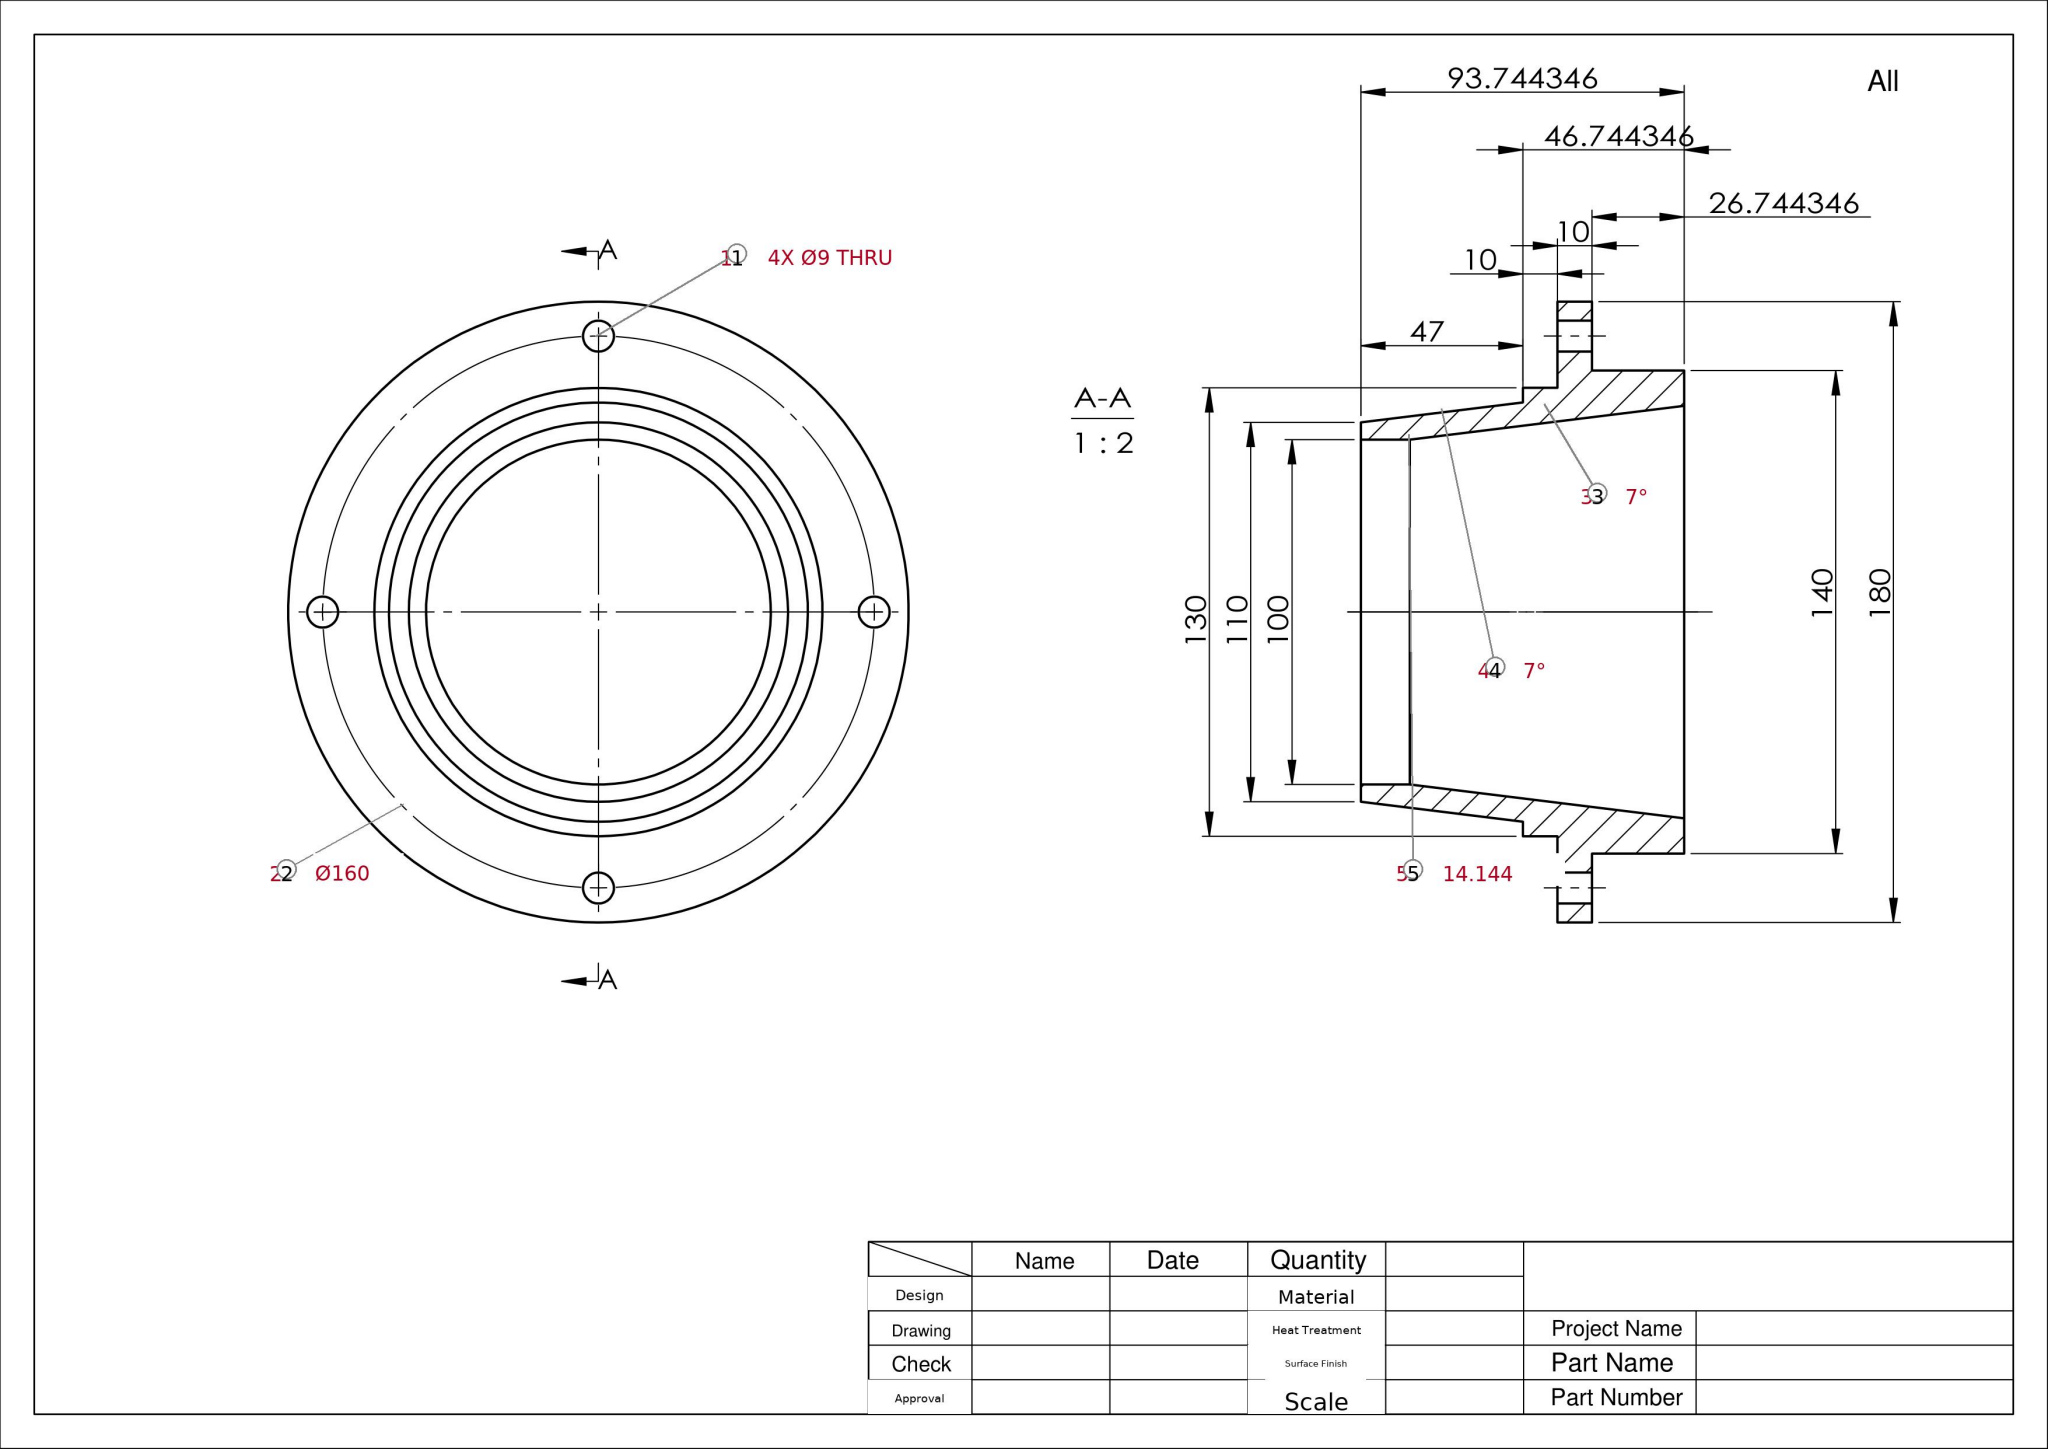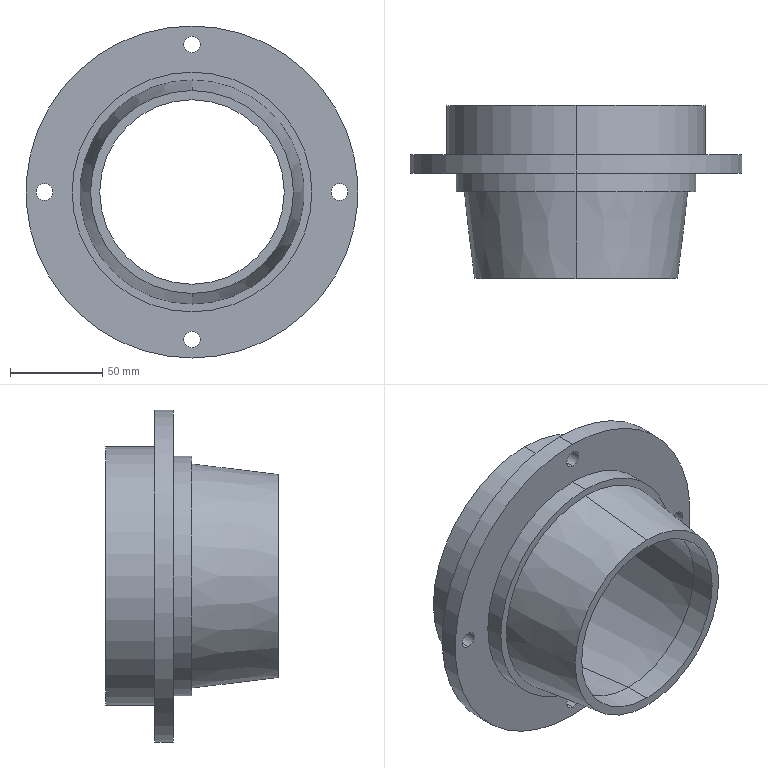Part | SolidWorks | mm | 1 solid | 25 faces | box 180 x 93.74 x 180 mm | volume 425080 mm3 | cylinder 16 | plane 5 | cone 4 | commonest cylinder face diameters 9 x8 180 x2 140 x2 100 x2 130 x2
STEP:
#1=CARTESIAN_POINT('',(0.,-6.,-55.));
#2=VERTEX_POINT('',#1);
#3=CARTESIAN_POINT('',(0.,-6.,55.));
#4=VERTEX_POINT('',#3);
#5=CARTESIAN_POINT('',(0.,-6.,0.));
#6=DIRECTION('',(0.,-1.,0.));
#7=DIRECTION('',(0.,0.,-1.));
#8=AXIS2_PLACEMENT_3D('',#5,#6,#7);
#9=CIRCLE('',#8,55.);
#10=EDGE_CURVE('',#2,#4,#9,.T.);
#11=ORIENTED_EDGE('',*,*,#10,.F.);
#12=CARTESIAN_POINT('',(0.,41.,-60.771));
#13=VERTEX_POINT('',#12);
#14=CARTESIAN_POINT('',(0.,41.,-60.771));
#15=DIRECTION('',(0.,0.9925,-0.1219));
#16=VECTOR('',#15,1000.);
#17=LINE('',#14,#16);
#18=EDGE_CURVE('',#2,#13,#17,.T.);
#19=ORIENTED_EDGE('',*,*,#18,.T.);
#20=CARTESIAN_POINT('',(0.,41.,60.771));
#21=VERTEX_POINT('',#20);
#22=CARTESIAN_POINT('',(0.,41.,0.));
#23=DIRECTION('',(0.,-1.,0.));
#24=DIRECTION('',(0.,0.,-1.));
#25=AXIS2_PLACEMENT_3D('',#22,#23,#24);
#26=CIRCLE('',#25,60.771);
#27=EDGE_CURVE('',#13,#21,#26,.T.);
#28=ORIENTED_EDGE('',*,*,#27,.T.);
#29=CARTESIAN_POINT('',(0.,41.,60.771));
#30=DIRECTION('',(0.,0.9925,0.1219));
#31=VECTOR('',#30,1000.);
#32=LINE('',#29,#31);
#33=EDGE_CURVE('',#4,#21,#32,.T.);
#34=ORIENTED_EDGE('',*,*,#33,.F.);
#35=EDGE_LOOP('',(#11,#19,#28,#34));
#36=FACE_OUTER_BOUND('',#35,.T.);
#37=CARTESIAN_POINT('',(0.,41.,0.));
#38=DIRECTION('',(0.,1.,0.));
#39=DIRECTION('',(0.,0.,1.));
#40=AXIS2_PLACEMENT_3D('',#37,#38,#39);
#41=CONICAL_SURFACE('',#40,60.771,0.1222);
#42=ADVANCED_FACE('',(#36),#41,.T.);
#43=CARTESIAN_POINT('',(80.,51.,4.5));
#44=VERTEX_POINT('',#43);
#45=CARTESIAN_POINT('',(80.,51.,-4.5));
#46=VERTEX_POINT('',#45);
#47=CARTESIAN_POINT('',(80.,51.,-0.));
#48=DIRECTION('',(0.,-1.,0.));
#49=DIRECTION('',(0.,0.,-1.));
#50=AXIS2_PLACEMENT_3D('',#47,#48,#49);
#51=CIRCLE('',#50,4.5);
#52=EDGE_CURVE('',#44,#46,#51,.T.);
#53=ORIENTED_EDGE('',*,*,#52,.T.);
#54=CARTESIAN_POINT('',(80.,61.,-4.5));
#55=VERTEX_POINT('',#54);
#56=CARTESIAN_POINT('',(80.,-10.,-4.5));
#57=DIRECTION('',(0.,1.,0.));
#58=VECTOR('',#57,1000.);
#59=LINE('',#56,#58);
#60=EDGE_CURVE('',#46,#55,#59,.T.);
#61=ORIENTED_EDGE('',*,*,#60,.T.);
#62=CARTESIAN_POINT('',(80.,61.,4.5));
#63=VERTEX_POINT('',#62);
#64=CARTESIAN_POINT('',(80.,61.,-0.));
#65=DIRECTION('',(0.,1.,0.));
#66=DIRECTION('',(-1.,0.,0.));
#67=AXIS2_PLACEMENT_3D('',#64,#65,#66);
#68=CIRCLE('',#67,4.5);
#69=EDGE_CURVE('',#55,#63,#68,.T.);
#70=ORIENTED_EDGE('',*,*,#69,.T.);
#71=CARTESIAN_POINT('',(80.,-10.,4.5));
#72=DIRECTION('',(0.,1.,0.));
#73=VECTOR('',#72,1000.);
#74=LINE('',#71,#73);
#75=EDGE_CURVE('',#44,#63,#74,.T.);
#76=ORIENTED_EDGE('',*,*,#75,.F.);
#77=EDGE_LOOP('',(#53,#61,#70,#76));
#78=FACE_OUTER_BOUND('',#77,.T.);
#79=CARTESIAN_POINT('',(80.,-10.,-0.));
#80=DIRECTION('',(0.,1.,0.));
#81=DIRECTION('',(0.,0.,1.));
#82=AXIS2_PLACEMENT_3D('',#79,#80,#81);
#83=CYLINDRICAL_SURFACE('',#82,4.5);
#84=ADVANCED_FACE('',(#78),#83,.F.);
#85=CARTESIAN_POINT('',(0.,51.,84.5));
#86=VERTEX_POINT('',#85);
#87=CARTESIAN_POINT('',(0.,51.,75.5));
#88=VERTEX_POINT('',#87);
#89=CARTESIAN_POINT('',(0.,51.,80.));
#90=DIRECTION('',(0.,-1.,0.));
#91=DIRECTION('',(0.,0.,-1.));
#92=AXIS2_PLACEMENT_3D('',#89,#90,#91);
#93=CIRCLE('',#92,4.5);
#94=EDGE_CURVE('',#86,#88,#93,.T.);
#95=ORIENTED_EDGE('',*,*,#94,.T.);
#96=CARTESIAN_POINT('',(0.,61.,75.5));
#97=VERTEX_POINT('',#96);
#98=CARTESIAN_POINT('',(0.,-10.,75.5));
#99=DIRECTION('',(0.,1.,0.));
#100=VECTOR('',#99,1000.);
#101=LINE('',#98,#100);
#102=EDGE_CURVE('',#88,#97,#101,.T.);
#103=ORIENTED_EDGE('',*,*,#102,.T.);
#104=CARTESIAN_POINT('',(0.,61.,84.5));
#105=VERTEX_POINT('',#104);
#106=CARTESIAN_POINT('',(0.,61.,80.));
#107=DIRECTION('',(0.,1.,0.));
#108=DIRECTION('',(-0.,0.,-1.));
#109=AXIS2_PLACEMENT_3D('',#106,#107,#108);
#110=CIRCLE('',#109,4.5);
#111=EDGE_CURVE('',#97,#105,#110,.T.);
#112=ORIENTED_EDGE('',*,*,#111,.T.);
#113=CARTESIAN_POINT('',(0.,-10.,84.5));
#114=DIRECTION('',(0.,1.,0.));
#115=VECTOR('',#114,1000.);
#116=LINE('',#113,#115);
#117=EDGE_CURVE('',#86,#105,#116,.T.);
#118=ORIENTED_EDGE('',*,*,#117,.F.);
#119=EDGE_LOOP('',(#95,#103,#112,#118));
#120=FACE_OUTER_BOUND('',#119,.T.);
#121=CARTESIAN_POINT('',(0.,-10.,80.));
#122=DIRECTION('',(0.,1.,0.));
#123=DIRECTION('',(0.,0.,1.));
#124=AXIS2_PLACEMENT_3D('',#121,#122,#123);
#125=CYLINDRICAL_SURFACE('',#124,4.5);
#126=ADVANCED_FACE('',(#120),#125,.F.);
#127=CARTESIAN_POINT('',(-80.,51.,4.5));
#128=VERTEX_POINT('',#127);
#129=CARTESIAN_POINT('',(-80.,51.,-4.5));
#130=VERTEX_POINT('',#129);
#131=CARTESIAN_POINT('',(-80.,51.,0.));
#132=DIRECTION('',(0.,-1.,0.));
#133=DIRECTION('',(0.,0.,-1.));
#134=AXIS2_PLACEMENT_3D('',#131,#132,#133);
#135=CIRCLE('',#134,4.5);
#136=EDGE_CURVE('',#128,#130,#135,.T.);
#137=ORIENTED_EDGE('',*,*,#136,.T.);
#138=CARTESIAN_POINT('',(-80.,61.,-4.5));
#139=VERTEX_POINT('',#138);
#140=CARTESIAN_POINT('',(-80.,-10.,-4.5));
#141=DIRECTION('',(0.,1.,0.));
#142=VECTOR('',#141,1000.);
#143=LINE('',#140,#142);
#144=EDGE_CURVE('',#130,#139,#143,.T.);
#145=ORIENTED_EDGE('',*,*,#144,.T.);
#146=CARTESIAN_POINT('',(-80.,61.,4.5));
#147=VERTEX_POINT('',#146);
#148=CARTESIAN_POINT('',(-80.,61.,0.));
#149=DIRECTION('',(0.,1.,0.));
#150=DIRECTION('',(1.,0.,-0.));
#151=AXIS2_PLACEMENT_3D('',#148,#149,#150);
#152=CIRCLE('',#151,4.5);
#153=EDGE_CURVE('',#139,#147,#152,.T.);
#154=ORIENTED_EDGE('',*,*,#153,.T.);
#155=CARTESIAN_POINT('',(-80.,-10.,4.5));
#156=DIRECTION('',(0.,1.,0.));
#157=VECTOR('',#156,1000.);
#158=LINE('',#155,#157);
#159=EDGE_CURVE('',#128,#147,#158,.T.);
#160=ORIENTED_EDGE('',*,*,#159,.F.);
#161=EDGE_LOOP('',(#137,#145,#154,#160));
#162=FACE_OUTER_BOUND('',#161,.T.);
#163=CARTESIAN_POINT('',(-80.,-10.,0.));
#164=DIRECTION('',(0.,1.,0.));
#165=DIRECTION('',(0.,0.,1.));
#166=AXIS2_PLACEMENT_3D('',#163,#164,#165);
#167=CYLINDRICAL_SURFACE('',#166,4.5);
#168=ADVANCED_FACE('',(#162),#167,.F.);
#169=CARTESIAN_POINT('',(0.,51.,-75.5));
#170=VERTEX_POINT('',#169);
#171=CARTESIAN_POINT('',(0.,51.,-84.5));
#172=VERTEX_POINT('',#171);
#173=CARTESIAN_POINT('',(0.,51.,-80.));
#174=DIRECTION('',(0.,-1.,0.));
#175=DIRECTION('',(0.,0.,-1.));
#176=AXIS2_PLACEMENT_3D('',#173,#174,#175);
#177=CIRCLE('',#176,4.5);
#178=EDGE_CURVE('',#170,#172,#177,.T.);
#179=ORIENTED_EDGE('',*,*,#178,.T.);
#180=CARTESIAN_POINT('',(0.,61.,-84.5));
#181=VERTEX_POINT('',#180);
#182=CARTESIAN_POINT('',(0.,-10.,-84.5));
#183=DIRECTION('',(0.,1.,0.));
#184=VECTOR('',#183,1000.);
#185=LINE('',#182,#184);
#186=EDGE_CURVE('',#172,#181,#185,.T.);
#187=ORIENTED_EDGE('',*,*,#186,.T.);
#188=CARTESIAN_POINT('',(0.,61.,-75.5));
#189=VERTEX_POINT('',#188);
#190=CARTESIAN_POINT('',(0.,61.,-80.));
#191=DIRECTION('',(0.,1.,0.));
#192=DIRECTION('',(0.,0.,1.));
#193=AXIS2_PLACEMENT_3D('',#190,#191,#192);
#194=CIRCLE('',#193,4.5);
#195=EDGE_CURVE('',#181,#189,#194,.T.);
#196=ORIENTED_EDGE('',*,*,#195,.T.);
#197=CARTESIAN_POINT('',(0.,-10.,-75.5));
#198=DIRECTION('',(0.,1.,0.));
#199=VECTOR('',#198,1000.);
#200=LINE('',#197,#199);
#201=EDGE_CURVE('',#170,#189,#200,.T.);
#202=ORIENTED_EDGE('',*,*,#201,.F.);
#203=EDGE_LOOP('',(#179,#187,#196,#202));
#204=FACE_OUTER_BOUND('',#203,.T.);
#205=CARTESIAN_POINT('',(0.,-10.,-80.));
#206=DIRECTION('',(0.,1.,0.));
#207=DIRECTION('',(0.,0.,1.));
#208=AXIS2_PLACEMENT_3D('',#205,#206,#207);
#209=CYLINDRICAL_SURFACE('',#208,4.5);
#210=ADVANCED_FACE('',(#204),#209,.F.);
#211=CARTESIAN_POINT('',(0.,51.,-90.));
#212=VERTEX_POINT('',#211);
#213=CARTESIAN_POINT('',(0.,51.,90.));
#214=VERTEX_POINT('',#213);
#215=CARTESIAN_POINT('',(0.,51.,0.));
#216=DIRECTION('',(0.,-1.,0.));
#217=DIRECTION('',(0.,0.,-1.));
#218=AXIS2_PLACEMENT_3D('',#215,#216,#217);
#219=CIRCLE('',#218,90.);
#220=EDGE_CURVE('',#212,#214,#219,.T.);
#221=ORIENTED_EDGE('',*,*,#220,.F.);
#222=CARTESIAN_POINT('',(0.,61.,-90.));
#223=VERTEX_POINT('',#222);
#224=CARTESIAN_POINT('',(0.,-10.,-90.));
#225=DIRECTION('',(0.,1.,0.));
#226=VECTOR('',#225,1000.);
#227=LINE('',#224,#226);
#228=EDGE_CURVE('',#212,#223,#227,.T.);
#229=ORIENTED_EDGE('',*,*,#228,.T.);
#230=CARTESIAN_POINT('',(0.,61.,90.));
#231=VERTEX_POINT('',#230);
#232=CARTESIAN_POINT('',(0.,61.,0.));
#233=DIRECTION('',(0.,1.,0.));
#234=DIRECTION('',(0.,0.,1.));
#235=AXIS2_PLACEMENT_3D('',#232,#233,#234);
#236=CIRCLE('',#235,90.);
#237=EDGE_CURVE('',#231,#223,#236,.T.);
#238=ORIENTED_EDGE('',*,*,#237,.F.);
#239=CARTESIAN_POINT('',(0.,-10.,90.));
#240=DIRECTION('',(0.,1.,0.));
#241=VECTOR('',#240,1000.);
#242=LINE('',#239,#241);
#243=EDGE_CURVE('',#214,#231,#242,.T.);
#244=ORIENTED_EDGE('',*,*,#243,.F.);
#245=EDGE_LOOP('',(#221,#229,#238,#244));
#246=FACE_OUTER_BOUND('',#245,.T.);
#247=CARTESIAN_POINT('',(0.,-10.,0.));
#248=DIRECTION('',(0.,1.,0.));
#249=DIRECTION('',(0.,0.,1.));
#250=AXIS2_PLACEMENT_3D('',#247,#248,#249);
#251=CYLINDRICAL_SURFACE('',#250,90.);
#252=ADVANCED_FACE('',(#246),#251,.T.);
#253=CARTESIAN_POINT('',(0.,61.,-70.));
#254=VERTEX_POINT('',#253);
#255=CARTESIAN_POINT('',(0.,61.,70.));
#256=VERTEX_POINT('',#255);
#257=CARTESIAN_POINT('',(0.,61.,0.));
#258=DIRECTION('',(0.,-1.,0.));
#259=DIRECTION('',(0.,0.,1.));
#260=AXIS2_PLACEMENT_3D('',#257,#258,#259);
#261=CIRCLE('',#260,70.);
#262=EDGE_CURVE('',#254,#256,#261,.T.);
#263=ORIENTED_EDGE('',*,*,#262,.F.);
#264=CARTESIAN_POINT('',(0.,87.744,-70.));
#265=VERTEX_POINT('',#264);
#266=CARTESIAN_POINT('',(0.,-191.367,-70.));
#267=DIRECTION('',(0.,1.,0.));
#268=VECTOR('',#267,1000.);
#269=LINE('',#266,#268);
#270=EDGE_CURVE('',#254,#265,#269,.T.);
#271=ORIENTED_EDGE('',*,*,#270,.T.);
#272=CARTESIAN_POINT('',(0.,87.744,70.));
#273=VERTEX_POINT('',#272);
#274=CARTESIAN_POINT('',(0.,87.744,0.));
#275=DIRECTION('',(0.,-1.,0.));
#276=DIRECTION('',(0.,0.,-1.));
#277=AXIS2_PLACEMENT_3D('',#274,#275,#276);
#278=CIRCLE('',#277,70.);
#279=EDGE_CURVE('',#265,#273,#278,.T.);
#280=ORIENTED_EDGE('',*,*,#279,.T.);
#281=CARTESIAN_POINT('',(0.,-191.367,70.));
#282=DIRECTION('',(0.,1.,0.));
#283=VECTOR('',#282,1000.);
#284=LINE('',#281,#283);
#285=EDGE_CURVE('',#256,#273,#284,.T.);
#286=ORIENTED_EDGE('',*,*,#285,.F.);
#287=EDGE_LOOP('',(#263,#271,#280,#286));
#288=FACE_OUTER_BOUND('',#287,.T.);
#289=CARTESIAN_POINT('',(0.,-191.367,0.));
#290=DIRECTION('',(0.,1.,0.));
#291=DIRECTION('',(0.,0.,1.));
#292=AXIS2_PLACEMENT_3D('',#289,#290,#291);
#293=CYLINDRICAL_SURFACE('',#292,70.);
#294=ADVANCED_FACE('',(#288),#293,.T.);
#295=CARTESIAN_POINT('',(0.,8.144,-50.));
#296=VERTEX_POINT('',#295);
#297=CARTESIAN_POINT('',(0.,8.144,50.));
#298=VERTEX_POINT('',#297);
#299=CARTESIAN_POINT('',(0.,8.144,0.));
#300=DIRECTION('',(0.,1.,0.));
#301=DIRECTION('',(0.,0.,1.));
#302=AXIS2_PLACEMENT_3D('',#299,#300,#301);
#303=CIRCLE('',#302,50.);
#304=EDGE_CURVE('',#296,#298,#303,.T.);
#305=ORIENTED_EDGE('',*,*,#304,.T.);
#306=CARTESIAN_POINT('',(0.,-6.,50.));
#307=VERTEX_POINT('',#306);
#308=CARTESIAN_POINT('',(0.,86.,50.));
#309=DIRECTION('',(0.,-1.,0.));
#310=VECTOR('',#309,1000.);
#311=LINE('',#308,#310);
#312=EDGE_CURVE('',#298,#307,#311,.T.);
#313=ORIENTED_EDGE('',*,*,#312,.T.);
#314=CARTESIAN_POINT('',(0.,-6.,-50.));
#315=VERTEX_POINT('',#314);
#316=CARTESIAN_POINT('',(0.,-6.,0.));
#317=DIRECTION('',(0.,-1.,0.));
#318=DIRECTION('',(0.,0.,1.));
#319=AXIS2_PLACEMENT_3D('',#316,#317,#318);
#320=CIRCLE('',#319,50.);
#321=EDGE_CURVE('',#307,#315,#320,.T.);
#322=ORIENTED_EDGE('',*,*,#321,.T.);
#323=CARTESIAN_POINT('',(0.,86.,-50.));
#324=DIRECTION('',(0.,-1.,0.));
#325=VECTOR('',#324,1000.);
#326=LINE('',#323,#325);
#327=EDGE_CURVE('',#296,#315,#326,.T.);
#328=ORIENTED_EDGE('',*,*,#327,.F.);
#329=EDGE_LOOP('',(#305,#313,#322,#328));
#330=FACE_OUTER_BOUND('',#329,.T.);
#331=CARTESIAN_POINT('',(0.,86.,0.));
#332=DIRECTION('',(0.,-1.,0.));
#333=DIRECTION('',(0.,0.,-1.));
#334=AXIS2_PLACEMENT_3D('',#331,#332,#333);
#335=CYLINDRICAL_SURFACE('',#334,50.);
#336=ADVANCED_FACE('',(#330),#335,.F.);
#337=CARTESIAN_POINT('',(0.,51.,-65.));
#338=VERTEX_POINT('',#337);
#339=CARTESIAN_POINT('',(0.,51.,65.));
#340=VERTEX_POINT('',#339);
#341=CARTESIAN_POINT('',(0.,51.,0.));
#342=DIRECTION('',(0.,-1.,0.));
#343=DIRECTION('',(0.,0.,-1.));
#344=AXIS2_PLACEMENT_3D('',#341,#342,#343);
#345=CIRCLE('',#344,65.);
#346=EDGE_CURVE('',#338,#340,#345,.T.);
#347=ORIENTED_EDGE('',*,*,#346,.T.);
#348=CARTESIAN_POINT('',(0.,41.,65.));
#349=VERTEX_POINT('',#348);
#350=CARTESIAN_POINT('',(0.,0.,65.));
#351=DIRECTION('',(0.,-1.,0.));
#352=VECTOR('',#351,1000.);
#353=LINE('',#350,#352);
#354=EDGE_CURVE('',#340,#349,#353,.T.);
#355=ORIENTED_EDGE('',*,*,#354,.T.);
#356=CARTESIAN_POINT('',(0.,41.,-65.));
#357=VERTEX_POINT('',#356);
#358=CARTESIAN_POINT('',(0.,41.,0.));
#359=DIRECTION('',(0.,-1.,0.));
#360=DIRECTION('',(0.,0.,-1.));
#361=AXIS2_PLACEMENT_3D('',#358,#359,#360);
#362=CIRCLE('',#361,65.);
#363=EDGE_CURVE('',#357,#349,#362,.T.);
#364=ORIENTED_EDGE('',*,*,#363,.F.);
#365=CARTESIAN_POINT('',(0.,0.,-65.));
#366=DIRECTION('',(0.,-1.,0.));
#367=VECTOR('',#366,1000.);
#368=LINE('',#365,#367);
#369=EDGE_CURVE('',#338,#357,#368,.T.);
#370=ORIENTED_EDGE('',*,*,#369,.F.);
#371=EDGE_LOOP('',(#347,#355,#364,#370));
#372=FACE_OUTER_BOUND('',#371,.T.);
#373=CARTESIAN_POINT('',(0.,0.,0.));
#374=DIRECTION('',(0.,-1.,0.));
#375=DIRECTION('',(0.,0.,-1.));
#376=AXIS2_PLACEMENT_3D('',#373,#374,#375);
#377=CYLINDRICAL_SURFACE('',#376,65.);
#378=ADVANCED_FACE('',(#372),#377,.T.);
#379=ORIENTED_EDGE('',*,*,#304,.F.);
#380=CARTESIAN_POINT('',(0.,87.744,-59.774));
#381=VERTEX_POINT('',#380);
#382=CARTESIAN_POINT('',(0.,86.,-59.559));
#383=DIRECTION('',(0.,0.9925,-0.1219));
#384=VECTOR('',#383,1000.);
#385=LINE('',#382,#384);
#386=EDGE_CURVE('',#296,#381,#385,.T.);
#387=ORIENTED_EDGE('',*,*,#386,.T.);
#388=CARTESIAN_POINT('',(0.,87.744,59.774));
#389=VERTEX_POINT('',#388);
#390=CARTESIAN_POINT('',(0.,87.744,0.));
#391=DIRECTION('',(0.,-1.,0.));
#392=DIRECTION('',(0.,0.,-1.));
#393=AXIS2_PLACEMENT_3D('',#390,#391,#392);
#394=CIRCLE('',#393,59.774);
#395=EDGE_CURVE('',#389,#381,#394,.T.);
#396=ORIENTED_EDGE('',*,*,#395,.F.);
#397=CARTESIAN_POINT('',(0.,86.,59.559));
#398=DIRECTION('',(0.,0.9925,0.1219));
#399=VECTOR('',#398,1000.);
#400=LINE('',#397,#399);
#401=EDGE_CURVE('',#298,#389,#400,.T.);
#402=ORIENTED_EDGE('',*,*,#401,.F.);
#403=EDGE_LOOP('',(#379,#387,#396,#402));
#404=FACE_OUTER_BOUND('',#403,.T.);
#405=CARTESIAN_POINT('',(0.,86.,0.));
#406=DIRECTION('',(0.,1.,0.));
#407=DIRECTION('',(0.,0.,1.));
#408=AXIS2_PLACEMENT_3D('',#405,#406,#407);
#409=CONICAL_SURFACE('',#408,59.559,0.1222);
#410=ADVANCED_FACE('',(#404),#409,.F.);
#411=ORIENTED_EDGE('',*,*,#52,.F.);
#412=CARTESIAN_POINT('',(80.,51.,-0.));
#413=DIRECTION('',(0.,-1.,0.));
#414=DIRECTION('',(0.,0.,-1.));
#415=AXIS2_PLACEMENT_3D('',#412,#413,#414);
#416=CIRCLE('',#415,4.5);
#417=EDGE_CURVE('',#46,#44,#416,.T.);
#418=ORIENTED_EDGE('',*,*,#417,.F.);
#419=EDGE_LOOP('',(#411,#418));
#420=FACE_BOUND('',#419,.T.);
#421=ORIENTED_EDGE('',*,*,#94,.F.);
#422=CARTESIAN_POINT('',(0.,51.,80.));
#423=DIRECTION('',(0.,-1.,0.));
#424=DIRECTION('',(0.,0.,-1.));
#425=AXIS2_PLACEMENT_3D('',#422,#423,#424);
#426=CIRCLE('',#425,4.5);
#427=EDGE_CURVE('',#88,#86,#426,.T.);
#428=ORIENTED_EDGE('',*,*,#427,.F.);
#429=EDGE_LOOP('',(#421,#428));
#430=FACE_BOUND('',#429,.T.);
#431=ORIENTED_EDGE('',*,*,#136,.F.);
#432=CARTESIAN_POINT('',(-80.,51.,0.));
#433=DIRECTION('',(0.,-1.,0.));
#434=DIRECTION('',(0.,0.,-1.));
#435=AXIS2_PLACEMENT_3D('',#432,#433,#434);
#436=CIRCLE('',#435,4.5);
#437=EDGE_CURVE('',#130,#128,#436,.T.);
#438=ORIENTED_EDGE('',*,*,#437,.F.);
#439=EDGE_LOOP('',(#431,#438));
#440=FACE_BOUND('',#439,.T.);
#441=ORIENTED_EDGE('',*,*,#178,.F.);
#442=CARTESIAN_POINT('',(0.,51.,-80.));
#443=DIRECTION('',(0.,-1.,0.));
#444=DIRECTION('',(0.,0.,-1.));
#445=AXIS2_PLACEMENT_3D('',#442,#443,#444);
#446=CIRCLE('',#445,4.5);
#447=EDGE_CURVE('',#172,#170,#446,.T.);
#448=ORIENTED_EDGE('',*,*,#447,.F.);
#449=EDGE_LOOP('',(#441,#448));
#450=FACE_BOUND('',#449,.T.);
#451=ORIENTED_EDGE('',*,*,#346,.F.);
#452=CARTESIAN_POINT('',(0.,51.,0.));
#453=DIRECTION('',(0.,-1.,0.));
#454=DIRECTION('',(0.,0.,-1.));
#455=AXIS2_PLACEMENT_3D('',#452,#453,#454);
#456=CIRCLE('',#455,65.);
#457=EDGE_CURVE('',#340,#338,#456,.T.);
#458=ORIENTED_EDGE('',*,*,#457,.F.);
#459=EDGE_LOOP('',(#451,#458));
#460=FACE_BOUND('',#459,.T.);
#461=CARTESIAN_POINT('',(0.,51.,0.));
#462=DIRECTION('',(0.,-1.,0.));
#463=DIRECTION('',(0.,0.,-1.));
#464=AXIS2_PLACEMENT_3D('',#461,#462,#463);
#465=CIRCLE('',#464,90.);
#466=EDGE_CURVE('',#214,#212,#465,.T.);
#467=ORIENTED_EDGE('',*,*,#466,.T.);
#468=ORIENTED_EDGE('',*,*,#220,.T.);
#469=EDGE_LOOP('',(#467,#468));
#470=FACE_OUTER_BOUND('',#469,.T.);
#471=CARTESIAN_POINT('',(110.,51.,0.));
#472=DIRECTION('',(0.,-1.,0.));
#473=DIRECTION('',(0.,0.,-1.));
#474=AXIS2_PLACEMENT_3D('',#471,#472,#473);
#475=PLANE('',#474);
#476=ADVANCED_FACE('',(#420,#430,#440,#450,#460,#470),#475,.T.);
#477=CARTESIAN_POINT('',(80.,61.,-0.));
#478=DIRECTION('',(0.,1.,0.));
#479=DIRECTION('',(-1.,0.,0.));
#480=AXIS2_PLACEMENT_3D('',#477,#478,#479);
#481=CIRCLE('',#480,4.5);
#482=EDGE_CURVE('',#63,#55,#481,.T.);
#483=ORIENTED_EDGE('',*,*,#482,.F.);
#484=ORIENTED_EDGE('',*,*,#69,.F.);
#485=EDGE_LOOP('',(#483,#484));
#486=FACE_BOUND('',#485,.T.);
#487=CARTESIAN_POINT('',(0.,61.,80.));
#488=DIRECTION('',(0.,1.,0.));
#489=DIRECTION('',(-0.,0.,-1.));
#490=AXIS2_PLACEMENT_3D('',#487,#488,#489);
#491=CIRCLE('',#490,4.5);
#492=EDGE_CURVE('',#105,#97,#491,.T.);
#493=ORIENTED_EDGE('',*,*,#492,.F.);
#494=ORIENTED_EDGE('',*,*,#111,.F.);
#495=EDGE_LOOP('',(#493,#494));
#496=FACE_BOUND('',#495,.T.);
#497=CARTESIAN_POINT('',(-80.,61.,0.));
#498=DIRECTION('',(0.,1.,0.));
#499=DIRECTION('',(1.,0.,-0.));
#500=AXIS2_PLACEMENT_3D('',#497,#498,#499);
#501=CIRCLE('',#500,4.5);
#502=EDGE_CURVE('',#147,#139,#501,.T.);
#503=ORIENTED_EDGE('',*,*,#502,.F.);
#504=ORIENTED_EDGE('',*,*,#153,.F.);
#505=EDGE_LOOP('',(#503,#504));
#506=FACE_BOUND('',#505,.T.);
#507=CARTESIAN_POINT('',(0.,61.,-80.));
#508=DIRECTION('',(0.,1.,0.));
#509=DIRECTION('',(0.,0.,1.));
#510=AXIS2_PLACEMENT_3D('',#507,#508,#509);
#511=CIRCLE('',#510,4.5);
#512=EDGE_CURVE('',#189,#181,#511,.T.);
#513=ORIENTED_EDGE('',*,*,#512,.F.);
#514=ORIENTED_EDGE('',*,*,#195,.F.);
#515=EDGE_LOOP('',(#513,#514));
#516=FACE_BOUND('',#515,.T.);
#517=CARTESIAN_POINT('',(0.,61.,0.));
#518=DIRECTION('',(0.,-1.,0.));
#519=DIRECTION('',(0.,0.,1.));
#520=AXIS2_PLACEMENT_3D('',#517,#518,#519);
#521=CIRCLE('',#520,70.);
#522=EDGE_CURVE('',#256,#254,#521,.T.);
#523=ORIENTED_EDGE('',*,*,#522,.T.);
#524=ORIENTED_EDGE('',*,*,#262,.T.);
#525=EDGE_LOOP('',(#523,#524));
#526=FACE_BOUND('',#525,.T.);
#527=ORIENTED_EDGE('',*,*,#237,.T.);
#528=CARTESIAN_POINT('',(0.,61.,0.));
#529=DIRECTION('',(0.,1.,0.));
#530=DIRECTION('',(0.,0.,1.));
#531=AXIS2_PLACEMENT_3D('',#528,#529,#530);
#532=CIRCLE('',#531,90.);
#533=EDGE_CURVE('',#223,#231,#532,.T.);
#534=ORIENTED_EDGE('',*,*,#533,.T.);
#535=EDGE_LOOP('',(#527,#534));
#536=FACE_OUTER_BOUND('',#535,.T.);
#537=CARTESIAN_POINT('',(0.,61.,0.));
#538=DIRECTION('',(0.,1.,0.));
#539=DIRECTION('',(0.,0.,1.));
#540=AXIS2_PLACEMENT_3D('',#537,#538,#539);
#541=PLANE('',#540);
#542=ADVANCED_FACE('',(#486,#496,#506,#516,#526,#536),#541,.T.);
#543=ORIENTED_EDGE('',*,*,#386,.F.);
#544=CARTESIAN_POINT('',(0.,8.144,0.));
#545=DIRECTION('',(0.,1.,0.));
#546=DIRECTION('',(0.,0.,1.));
#547=AXIS2_PLACEMENT_3D('',#544,#545,#546);
#548=CIRCLE('',#547,50.);
#549=EDGE_CURVE('',#298,#296,#548,.T.);
#550=ORIENTED_EDGE('',*,*,#549,.F.);
#551=ORIENTED_EDGE('',*,*,#401,.T.);
#552=CARTESIAN_POINT('',(0.,87.744,0.));
#553=DIRECTION('',(0.,-1.,0.));
#554=DIRECTION('',(0.,0.,-1.));
#555=AXIS2_PLACEMENT_3D('',#552,#553,#554);
#556=CIRCLE('',#555,59.774);
#557=EDGE_CURVE('',#381,#389,#556,.T.);
#558=ORIENTED_EDGE('',*,*,#557,.F.);
#559=EDGE_LOOP('',(#543,#550,#551,#558));
#560=FACE_OUTER_BOUND('',#559,.T.);
#561=CARTESIAN_POINT('',(0.,86.,0.));
#562=DIRECTION('',(0.,1.,0.));
#563=DIRECTION('',(0.,0.,1.));
#564=AXIS2_PLACEMENT_3D('',#561,#562,#563);
#565=CONICAL_SURFACE('',#564,59.559,0.1222);
#566=ADVANCED_FACE('',(#560),#565,.F.);
#567=ORIENTED_EDGE('',*,*,#354,.F.);
#568=ORIENTED_EDGE('',*,*,#457,.T.);
#569=ORIENTED_EDGE('',*,*,#369,.T.);
#570=CARTESIAN_POINT('',(0.,41.,0.));
#571=DIRECTION('',(0.,-1.,0.));
#572=DIRECTION('',(0.,0.,-1.));
#573=AXIS2_PLACEMENT_3D('',#570,#571,#572);
#574=CIRCLE('',#573,65.);
#575=EDGE_CURVE('',#349,#357,#574,.T.);
#576=ORIENTED_EDGE('',*,*,#575,.F.);
#577=EDGE_LOOP('',(#567,#568,#569,#576));
#578=FACE_OUTER_BOUND('',#577,.T.);
#579=CARTESIAN_POINT('',(0.,0.,0.));
#580=DIRECTION('',(0.,-1.,0.));
#581=DIRECTION('',(0.,0.,-1.));
#582=AXIS2_PLACEMENT_3D('',#579,#580,#581);
#583=CYLINDRICAL_SURFACE('',#582,65.);
#584=ADVANCED_FACE('',(#578),#583,.T.);
#585=ORIENTED_EDGE('',*,*,#312,.F.);
#586=ORIENTED_EDGE('',*,*,#549,.T.);
#587=ORIENTED_EDGE('',*,*,#327,.T.);
#588=CARTESIAN_POINT('',(0.,-6.,0.));
#589=DIRECTION('',(0.,-1.,0.));
#590=DIRECTION('',(0.,0.,1.));
#591=AXIS2_PLACEMENT_3D('',#588,#589,#590);
#592=CIRCLE('',#591,50.);
#593=EDGE_CURVE('',#315,#307,#592,.T.);
#594=ORIENTED_EDGE('',*,*,#593,.T.);
#595=EDGE_LOOP('',(#585,#586,#587,#594));
#596=FACE_OUTER_BOUND('',#595,.T.);
#597=CARTESIAN_POINT('',(0.,86.,0.));
#598=DIRECTION('',(0.,-1.,0.));
#599=DIRECTION('',(0.,0.,-1.));
#600=AXIS2_PLACEMENT_3D('',#597,#598,#599);
#601=CYLINDRICAL_SURFACE('',#600,50.);
#602=ADVANCED_FACE('',(#596),#601,.F.);
#603=ORIENTED_EDGE('',*,*,#270,.F.);
#604=ORIENTED_EDGE('',*,*,#522,.F.);
#605=ORIENTED_EDGE('',*,*,#285,.T.);
#606=CARTESIAN_POINT('',(0.,87.744,0.));
#607=DIRECTION('',(0.,-1.,0.));
#608=DIRECTION('',(0.,0.,-1.));
#609=AXIS2_PLACEMENT_3D('',#606,#607,#608);
#610=CIRCLE('',#609,70.);
#611=EDGE_CURVE('',#273,#265,#610,.T.);
#612=ORIENTED_EDGE('',*,*,#611,.T.);
#613=EDGE_LOOP('',(#603,#604,#605,#612));
#614=FACE_OUTER_BOUND('',#613,.T.);
#615=CARTESIAN_POINT('',(0.,-191.367,0.));
#616=DIRECTION('',(0.,1.,0.));
#617=DIRECTION('',(0.,0.,1.));
#618=AXIS2_PLACEMENT_3D('',#615,#616,#617);
#619=CYLINDRICAL_SURFACE('',#618,70.);
#620=ADVANCED_FACE('',(#614),#619,.T.);
#621=ORIENTED_EDGE('',*,*,#228,.F.);
#622=ORIENTED_EDGE('',*,*,#466,.F.);
#623=ORIENTED_EDGE('',*,*,#243,.T.);
#624=ORIENTED_EDGE('',*,*,#533,.F.);
#625=EDGE_LOOP('',(#621,#622,#623,#624));
#626=FACE_OUTER_BOUND('',#625,.T.);
#627=CARTESIAN_POINT('',(0.,-10.,0.));
#628=DIRECTION('',(0.,1.,0.));
#629=DIRECTION('',(0.,0.,1.));
#630=AXIS2_PLACEMENT_3D('',#627,#628,#629);
#631=CYLINDRICAL_SURFACE('',#630,90.);
#632=ADVANCED_FACE('',(#626),#631,.T.);
#633=ORIENTED_EDGE('',*,*,#186,.F.);
#634=ORIENTED_EDGE('',*,*,#447,.T.);
#635=ORIENTED_EDGE('',*,*,#201,.T.);
#636=ORIENTED_EDGE('',*,*,#512,.T.);
#637=EDGE_LOOP('',(#633,#634,#635,#636));
#638=FACE_OUTER_BOUND('',#637,.T.);
#639=CARTESIAN_POINT('',(0.,-10.,-80.));
#640=DIRECTION('',(0.,1.,0.));
#641=DIRECTION('',(0.,0.,1.));
#642=AXIS2_PLACEMENT_3D('',#639,#640,#641);
#643=CYLINDRICAL_SURFACE('',#642,4.5);
#644=ADVANCED_FACE('',(#638),#643,.F.);
#645=ORIENTED_EDGE('',*,*,#144,.F.);
#646=ORIENTED_EDGE('',*,*,#437,.T.);
#647=ORIENTED_EDGE('',*,*,#159,.T.);
#648=ORIENTED_EDGE('',*,*,#502,.T.);
#649=EDGE_LOOP('',(#645,#646,#647,#648));
#650=FACE_OUTER_BOUND('',#649,.T.);
#651=CARTESIAN_POINT('',(-80.,-10.,0.));
#652=DIRECTION('',(0.,1.,0.));
#653=DIRECTION('',(0.,0.,1.));
#654=AXIS2_PLACEMENT_3D('',#651,#652,#653);
#655=CYLINDRICAL_SURFACE('',#654,4.5);
#656=ADVANCED_FACE('',(#650),#655,.F.);
#657=ORIENTED_EDGE('',*,*,#102,.F.);
#658=ORIENTED_EDGE('',*,*,#427,.T.);
#659=ORIENTED_EDGE('',*,*,#117,.T.);
#660=ORIENTED_EDGE('',*,*,#492,.T.);
#661=EDGE_LOOP('',(#657,#658,#659,#660));
#662=FACE_OUTER_BOUND('',#661,.T.);
#663=CARTESIAN_POINT('',(0.,-10.,80.));
#664=DIRECTION('',(0.,1.,0.));
#665=DIRECTION('',(0.,0.,1.));
#666=AXIS2_PLACEMENT_3D('',#663,#664,#665);
#667=CYLINDRICAL_SURFACE('',#666,4.5);
#668=ADVANCED_FACE('',(#662),#667,.F.);
#669=ORIENTED_EDGE('',*,*,#60,.F.);
#670=ORIENTED_EDGE('',*,*,#417,.T.);
#671=ORIENTED_EDGE('',*,*,#75,.T.);
#672=ORIENTED_EDGE('',*,*,#482,.T.);
#673=EDGE_LOOP('',(#669,#670,#671,#672));
#674=FACE_OUTER_BOUND('',#673,.T.);
#675=CARTESIAN_POINT('',(80.,-10.,-0.));
#676=DIRECTION('',(0.,1.,0.));
#677=DIRECTION('',(0.,0.,1.));
#678=AXIS2_PLACEMENT_3D('',#675,#676,#677);
#679=CYLINDRICAL_SURFACE('',#678,4.5);
#680=ADVANCED_FACE('',(#674),#679,.F.);
#681=CARTESIAN_POINT('',(0.,-6.,0.));
#682=DIRECTION('',(0.,-1.,0.));
#683=DIRECTION('',(0.,0.,-1.));
#684=AXIS2_PLACEMENT_3D('',#681,#682,#683);
#685=CIRCLE('',#684,55.);
#686=EDGE_CURVE('',#4,#2,#685,.T.);
#687=ORIENTED_EDGE('',*,*,#686,.T.);
#688=ORIENTED_EDGE('',*,*,#10,.T.);
#689=EDGE_LOOP('',(#687,#688));
#690=FACE_OUTER_BOUND('',#689,.T.);
#691=ORIENTED_EDGE('',*,*,#593,.F.);
#692=ORIENTED_EDGE('',*,*,#321,.F.);
#693=EDGE_LOOP('',(#691,#692));
#694=FACE_BOUND('',#693,.T.);
#695=CARTESIAN_POINT('',(0.,-6.,-18.544));
#696=DIRECTION('',(0.,1.,0.));
#697=DIRECTION('',(0.,0.,1.));
#698=AXIS2_PLACEMENT_3D('',#695,#696,#697);
#699=PLANE('',#698);
#700=ADVANCED_FACE('',(#690,#694),#699,.F.);
#701=CARTESIAN_POINT('',(0.,41.,0.));
#702=DIRECTION('',(0.,-1.,0.));
#703=DIRECTION('',(0.,0.,-1.));
#704=AXIS2_PLACEMENT_3D('',#701,#702,#703);
#705=CIRCLE('',#704,60.771);
#706=EDGE_CURVE('',#21,#13,#705,.T.);
#707=ORIENTED_EDGE('',*,*,#706,.F.);
#708=ORIENTED_EDGE('',*,*,#27,.F.);
#709=EDGE_LOOP('',(#707,#708));
#710=FACE_BOUND('',#709,.T.);
#711=ORIENTED_EDGE('',*,*,#363,.T.);
#712=ORIENTED_EDGE('',*,*,#575,.T.);
#713=EDGE_LOOP('',(#711,#712));
#714=FACE_OUTER_BOUND('',#713,.T.);
#715=CARTESIAN_POINT('',(0.,41.,-65.));
#716=DIRECTION('',(0.,1.,0.));
#717=DIRECTION('',(0.,0.,1.));
#718=AXIS2_PLACEMENT_3D('',#715,#716,#717);
#719=PLANE('',#718);
#720=ADVANCED_FACE('',(#710,#714),#719,.F.);
#721=ORIENTED_EDGE('',*,*,#18,.F.);
#722=ORIENTED_EDGE('',*,*,#686,.F.);
#723=ORIENTED_EDGE('',*,*,#33,.T.);
#724=ORIENTED_EDGE('',*,*,#706,.T.);
#725=EDGE_LOOP('',(#721,#722,#723,#724));
#726=FACE_OUTER_BOUND('',#725,.T.);
#727=CARTESIAN_POINT('',(0.,41.,0.));
#728=DIRECTION('',(0.,1.,0.));
#729=DIRECTION('',(0.,0.,1.));
#730=AXIS2_PLACEMENT_3D('',#727,#728,#729);
#731=CONICAL_SURFACE('',#730,60.771,0.1222);
#732=ADVANCED_FACE('',(#726),#731,.T.);
#733=ORIENTED_EDGE('',*,*,#611,.F.);
#734=ORIENTED_EDGE('',*,*,#279,.F.);
#735=EDGE_LOOP('',(#733,#734));
#736=FACE_OUTER_BOUND('',#735,.T.);
#737=ORIENTED_EDGE('',*,*,#395,.T.);
#738=ORIENTED_EDGE('',*,*,#557,.T.);
#739=EDGE_LOOP('',(#737,#738));
#740=FACE_BOUND('',#739,.T.);
#741=CARTESIAN_POINT('',(0.,87.744,59.774));
#742=DIRECTION('',(0.,-1.,0.));
#743=DIRECTION('',(0.,0.,-1.));
#744=AXIS2_PLACEMENT_3D('',#741,#742,#743);
#745=PLANE('',#744);
#746=ADVANCED_FACE('',(#736,#740),#745,.F.);
#747=CLOSED_SHELL('',(#42,#84,#126,#168,#210,#252,#294,#336,#378,#410,#476,#542,#566,#584,#602,#620,#632,#644,#656,#668,#680,#700,#720,#732,#746));
#748=MANIFOLD_SOLID_BREP('',#747);
#749=CARTESIAN_POINT('',(0.,0.,0.));
#750=DIRECTION('',(0.,0.,1.));
#751=DIRECTION('',(1.,0.,0.));
#752=AXIS2_PLACEMENT_3D('',#749,#750,#751);
#753=(LENGTH_UNIT()NAMED_UNIT(*)SI_UNIT(.MILLI.,.METRE.));
#754=UNCERTAINTY_MEASURE_WITH_UNIT(LENGTH_MEASURE(0.00001),#753,'','');
#755=(NAMED_UNIT(*)PLANE_ANGLE_UNIT()SI_UNIT($,.RADIAN.));
#756=(NAMED_UNIT(*)SI_UNIT($,.STERADIAN.)SOLID_ANGLE_UNIT());
#757=(GEOMETRIC_REPRESENTATION_CONTEXT(3)GLOBAL_UNCERTAINTY_ASSIGNED_CONTEXT((#754))GLOBAL_UNIT_ASSIGNED_CONTEXT((#753,#755,#756))REPRESENTATION_CONTEXT('',''));
#758=ADVANCED_BREP_SHAPE_REPRESENTATION('',(#748,#752),#757);